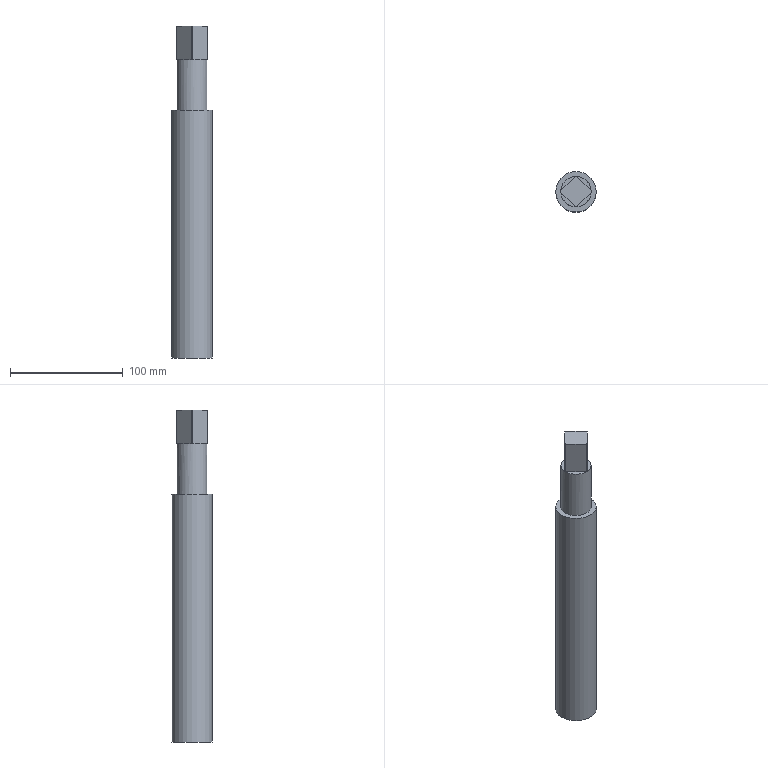Component | NX | SCREW_ROD | 1 solid | 16 faces | box 36 x 36 x 295 mm | volume 260111 mm3 | plane 12 | cylinder 3 | cone 1 | commonest cylinder face diameters 36 x1 27 x1 9.732 x1
STEP:
#1=CARTESIAN_POINT('',(0.,0.,0.));
#2=DIRECTION('',(0.,0.,1.));
#3=DIRECTION('',(1.,0.,0.));
#4=AXIS2_PLACEMENT_3D('',#1,#2,#3);
#5=CARTESIAN_POINT('',(18.,-0.,142.5));
#6=VERTEX_POINT('',#5);
#7=CARTESIAN_POINT('',(-0.,-0.,142.5));
#8=DIRECTION('',(0.,0.,1.));
#9=DIRECTION('',(1.,0.,0.));
#10=AXIS2_PLACEMENT_3D('',#7,#8,#9);
#11=CIRCLE('',#10,18.);
#12=CARTESIAN_POINT('',(-0.,-0.,142.5));
#13=DIRECTION('',(0.,0.,-1.));
#14=DIRECTION('',(-1.,0.,0.));
#15=AXIS2_PLACEMENT_3D('',#12,#13,#14);
#16=CYLINDRICAL_SURFACE('',#15,18.);
#17=CARTESIAN_POINT('',(9.425,0.));
#18=DIRECTION('',(-1.,0.));
#19=VECTOR('',#18,1.);
#20=LINE('',#17,#19);
#21=(GEOMETRIC_REPRESENTATION_CONTEXT(2)PARAMETRIC_REPRESENTATION_CONTEXT()REPRESENTATION_CONTEXT('',''));
#22=DEFINITIONAL_REPRESENTATION('',(#20),#21);
#23=PCURVE('',#16,#22);
#24=CARTESIAN_POINT('',(-0.,-0.,142.5));
#25=DIRECTION('',(0.,0.,1.));
#26=DIRECTION('',(1.,0.,0.));
#27=AXIS2_PLACEMENT_3D('',#24,#25,#26);
#28=PLANE('',#27);
#29=CARTESIAN_POINT('',(0.,0.));
#30=DIRECTION('',(1.,0.));
#31=AXIS2_PLACEMENT_2D('',#29,#30);
#32=CIRCLE('',#31,18.);
#33=(GEOMETRIC_REPRESENTATION_CONTEXT(2)PARAMETRIC_REPRESENTATION_CONTEXT()REPRESENTATION_CONTEXT('',''));
#34=DEFINITIONAL_REPRESENTATION('',(#32),#33);
#35=PCURVE('',#28,#34);
#36=SURFACE_CURVE('',#11,(#23,#35),.PCURVE_S1.);
#37=EDGE_CURVE('',#6,#6,#36,.T.);
#38=ORIENTED_EDGE('',*,*,#37,.F.);
#39=CARTESIAN_POINT('',(18.,-0.,-77.5));
#40=VERTEX_POINT('',#39);
#41=CARTESIAN_POINT('',(18.,-0.,142.5));
#42=CARTESIAN_POINT('',(18.,-0.,-77.5));
#43=B_SPLINE_CURVE_WITH_KNOTS('',1,(#41,#42),.UNSPECIFIED.,.F.,.F.,(2,2),(0.,220.),.PIECEWISE_BEZIER_KNOTS.);
#44=CARTESIAN_POINT('',(9.425,0.));
#45=DIRECTION('',(0.,1.));
#46=VECTOR('',#45,1.);
#47=LINE('',#44,#46);
#48=(GEOMETRIC_REPRESENTATION_CONTEXT(2)PARAMETRIC_REPRESENTATION_CONTEXT()REPRESENTATION_CONTEXT('',''));
#49=DEFINITIONAL_REPRESENTATION('',(#47),#48);
#50=PCURVE('',#16,#49);
#51=CARTESIAN_POINT('',(3.142,0.));
#52=DIRECTION('',(0.,1.));
#53=VECTOR('',#52,1.);
#54=LINE('',#51,#53);
#55=(GEOMETRIC_REPRESENTATION_CONTEXT(2)PARAMETRIC_REPRESENTATION_CONTEXT()REPRESENTATION_CONTEXT('',''));
#56=DEFINITIONAL_REPRESENTATION('',(#54),#55);
#57=PCURVE('',#16,#56);
#58=SEAM_CURVE('',#43,(#50,#57),.PCURVE_S1.);
#59=EDGE_CURVE('',#6,#40,#58,.T.);
#60=ORIENTED_EDGE('',*,*,#59,.T.);
#61=CARTESIAN_POINT('',(-0.,-0.,-77.5));
#62=DIRECTION('',(0.,0.,1.));
#63=DIRECTION('',(1.,0.,0.));
#64=AXIS2_PLACEMENT_3D('',#61,#62,#63);
#65=CIRCLE('',#64,18.);
#66=CARTESIAN_POINT('',(9.425,220.));
#67=DIRECTION('',(-1.,0.));
#68=VECTOR('',#67,1.);
#69=LINE('',#66,#68);
#70=(GEOMETRIC_REPRESENTATION_CONTEXT(2)PARAMETRIC_REPRESENTATION_CONTEXT()REPRESENTATION_CONTEXT('',''));
#71=DEFINITIONAL_REPRESENTATION('',(#69),#70);
#72=PCURVE('',#16,#71);
#73=CARTESIAN_POINT('',(-0.,-0.,-77.5));
#74=DIRECTION('',(0.,0.,1.));
#75=DIRECTION('',(1.,0.,0.));
#76=AXIS2_PLACEMENT_3D('',#73,#74,#75);
#77=PLANE('',#76);
#78=CARTESIAN_POINT('',(0.,0.));
#79=DIRECTION('',(1.,0.));
#80=AXIS2_PLACEMENT_2D('',#78,#79);
#81=CIRCLE('',#80,18.);
#82=(GEOMETRIC_REPRESENTATION_CONTEXT(2)PARAMETRIC_REPRESENTATION_CONTEXT()REPRESENTATION_CONTEXT('',''));
#83=DEFINITIONAL_REPRESENTATION('',(#81),#82);
#84=PCURVE('',#77,#83);
#85=SURFACE_CURVE('',#65,(#72,#84),.PCURVE_S1.);
#86=EDGE_CURVE('',#40,#40,#85,.T.);
#87=ORIENTED_EDGE('',*,*,#86,.T.);
#88=ORIENTED_EDGE('',*,*,#59,.F.);
#89=EDGE_LOOP('',(#38,#60,#87,#88));
#90=FACE_BOUND('',#89,.T.);
#91=ADVANCED_FACE('',(#90),#16,.T.);
#92=CARTESIAN_POINT('',(13.5,-0.,142.5));
#93=VERTEX_POINT('',#92);
#94=CARTESIAN_POINT('',(-13.484,-0.6582,142.5));
#95=VERTEX_POINT('',#94);
#96=CARTESIAN_POINT('',(-0.,-0.,142.5));
#97=DIRECTION('',(0.,0.,1.));
#98=DIRECTION('',(1.,0.,0.));
#99=AXIS2_PLACEMENT_3D('',#96,#97,#98);
#100=CIRCLE('',#99,13.5);
#101=CARTESIAN_POINT('',(0.,0.));
#102=DIRECTION('',(1.,0.));
#103=AXIS2_PLACEMENT_2D('',#101,#102);
#104=CIRCLE('',#103,13.5);
#105=(GEOMETRIC_REPRESENTATION_CONTEXT(2)PARAMETRIC_REPRESENTATION_CONTEXT()REPRESENTATION_CONTEXT('',''));
#106=DEFINITIONAL_REPRESENTATION('',(#104),#105);
#107=PCURVE('',#28,#106);
#108=CARTESIAN_POINT('',(-0.,-0.,217.5));
#109=DIRECTION('',(0.,0.,-1.));
#110=DIRECTION('',(-1.,0.,0.));
#111=AXIS2_PLACEMENT_3D('',#108,#109,#110);
#112=CYLINDRICAL_SURFACE('',#111,13.5);
#113=CARTESIAN_POINT('',(9.425,75.));
#114=DIRECTION('',(-1.,0.));
#115=VECTOR('',#114,1.);
#116=LINE('',#113,#115);
#117=(GEOMETRIC_REPRESENTATION_CONTEXT(2)PARAMETRIC_REPRESENTATION_CONTEXT()REPRESENTATION_CONTEXT('',''));
#118=DEFINITIONAL_REPRESENTATION('',(#116),#117);
#119=PCURVE('',#112,#118);
#120=SURFACE_CURVE('',#100,(#107,#119),.PCURVE_S1.);
#121=EDGE_CURVE('',#93,#95,#120,.T.);
#122=ORIENTED_EDGE('',*,*,#121,.F.);
#123=CARTESIAN_POINT('',(-0.,-0.,142.5));
#124=DIRECTION('',(0.,0.,1.));
#125=DIRECTION('',(1.,0.,0.));
#126=AXIS2_PLACEMENT_3D('',#123,#124,#125);
#127=CIRCLE('',#126,13.5);
#128=CARTESIAN_POINT('',(0.,0.));
#129=DIRECTION('',(1.,0.));
#130=AXIS2_PLACEMENT_2D('',#128,#129);
#131=CIRCLE('',#130,13.5);
#132=(GEOMETRIC_REPRESENTATION_CONTEXT(2)PARAMETRIC_REPRESENTATION_CONTEXT()REPRESENTATION_CONTEXT('',''));
#133=DEFINITIONAL_REPRESENTATION('',(#131),#132);
#134=PCURVE('',#28,#133);
#135=CARTESIAN_POINT('',(15.708,75.));
#136=DIRECTION('',(-1.,0.));
#137=VECTOR('',#136,1.);
#138=LINE('',#135,#137);
#139=(GEOMETRIC_REPRESENTATION_CONTEXT(2)PARAMETRIC_REPRESENTATION_CONTEXT()REPRESENTATION_CONTEXT('',''));
#140=DEFINITIONAL_REPRESENTATION('',(#138),#139);
#141=PCURVE('',#112,#140);
#142=SURFACE_CURVE('',#127,(#134,#141),.PCURVE_S1.);
#143=EDGE_CURVE('',#95,#93,#142,.T.);
#144=ORIENTED_EDGE('',*,*,#143,.F.);
#145=EDGE_LOOP('',(#122,#144));
#146=FACE_BOUND('',#145,.T.);
#147=ORIENTED_EDGE('',*,*,#37,.T.);
#148=EDGE_LOOP('',(#147));
#149=FACE_BOUND('',#148,.T.);
#150=ADVANCED_FACE('',(#146,#149),#28,.T.);
#151=CARTESIAN_POINT('',(4.866,-0.,-77.5));
#152=VERTEX_POINT('',#151);
#153=CARTESIAN_POINT('',(-0.,-0.,-77.5));
#154=DIRECTION('',(0.,0.,1.));
#155=DIRECTION('',(1.,0.,0.));
#156=AXIS2_PLACEMENT_3D('',#153,#154,#155);
#157=CIRCLE('',#156,4.866);
#158=CARTESIAN_POINT('',(0.,0.));
#159=DIRECTION('',(1.,0.));
#160=AXIS2_PLACEMENT_2D('',#158,#159);
#161=CIRCLE('',#160,4.866);
#162=(GEOMETRIC_REPRESENTATION_CONTEXT(2)PARAMETRIC_REPRESENTATION_CONTEXT()REPRESENTATION_CONTEXT('',''));
#163=DEFINITIONAL_REPRESENTATION('',(#161),#162);
#164=PCURVE('',#77,#163);
#165=CARTESIAN_POINT('',(-0.,-0.,-78.5));
#166=DIRECTION('',(0.,0.,1.));
#167=DIRECTION('',(1.,0.,0.));
#168=AXIS2_PLACEMENT_3D('',#165,#166,#167);
#169=CYLINDRICAL_SURFACE('',#168,4.866);
#170=CARTESIAN_POINT('',(0.,1.));
#171=DIRECTION('',(1.,0.));
#172=VECTOR('',#171,1.);
#173=LINE('',#170,#172);
#174=(GEOMETRIC_REPRESENTATION_CONTEXT(2)PARAMETRIC_REPRESENTATION_CONTEXT()REPRESENTATION_CONTEXT('',''));
#175=DEFINITIONAL_REPRESENTATION('',(#173),#174);
#176=PCURVE('',#169,#175);
#177=SURFACE_CURVE('',#157,(#164,#176),.PCURVE_S1.);
#178=EDGE_CURVE('',#152,#152,#177,.T.);
#179=ORIENTED_EDGE('',*,*,#178,.T.);
#180=EDGE_LOOP('',(#179));
#181=FACE_BOUND('',#180,.T.);
#182=ORIENTED_EDGE('',*,*,#86,.F.);
#183=EDGE_LOOP('',(#182));
#184=FACE_BOUND('',#183,.T.);
#185=ADVANCED_FACE('',(#181,#184),#77,.F.);
#186=CARTESIAN_POINT('',(-0.6582,-13.484,217.5));
#187=VERTEX_POINT('',#186);
#188=CARTESIAN_POINT('',(0.6582,-13.484,217.5));
#189=VERTEX_POINT('',#188);
#190=CARTESIAN_POINT('',(-0.,-0.,217.5));
#191=DIRECTION('',(0.,0.,1.));
#192=DIRECTION('',(1.,0.,0.));
#193=AXIS2_PLACEMENT_3D('',#190,#191,#192);
#194=CIRCLE('',#193,13.5);
#195=CARTESIAN_POINT('',(15.708,0.));
#196=DIRECTION('',(-1.,0.));
#197=VECTOR('',#196,1.);
#198=LINE('',#195,#197);
#199=(GEOMETRIC_REPRESENTATION_CONTEXT(2)PARAMETRIC_REPRESENTATION_CONTEXT()REPRESENTATION_CONTEXT('',''));
#200=DEFINITIONAL_REPRESENTATION('',(#198),#199);
#201=PCURVE('',#112,#200);
#202=CARTESIAN_POINT('',(-0.,-0.,217.5));
#203=DIRECTION('',(0.,0.,1.));
#204=DIRECTION('',(1.,0.,0.));
#205=AXIS2_PLACEMENT_3D('',#202,#203,#204);
#206=PLANE('',#205);
#207=CARTESIAN_POINT('',(0.,0.));
#208=DIRECTION('',(1.,0.));
#209=AXIS2_PLACEMENT_2D('',#207,#208);
#210=CIRCLE('',#209,13.5);
#211=(GEOMETRIC_REPRESENTATION_CONTEXT(2)PARAMETRIC_REPRESENTATION_CONTEXT()REPRESENTATION_CONTEXT('',''));
#212=DEFINITIONAL_REPRESENTATION('',(#210),#211);
#213=PCURVE('',#206,#212);
#214=SURFACE_CURVE('',#194,(#201,#213),.PCURVE_S1.);
#215=EDGE_CURVE('',#187,#189,#214,.T.);
#216=ORIENTED_EDGE('',*,*,#215,.F.);
#217=CARTESIAN_POINT('',(-0.6582,-13.484,187.5));
#218=VERTEX_POINT('',#217);
#219=CARTESIAN_POINT('',(-0.6582,-13.484,187.5));
#220=DIRECTION('',(0.,0.,-1.));
#221=VECTOR('',#220,1.);
#222=LINE('',#219,#221);
#223=CARTESIAN_POINT('',(11.044,30.));
#224=DIRECTION('',(0.,1.));
#225=VECTOR('',#224,1.);
#226=LINE('',#223,#225);
#227=(GEOMETRIC_REPRESENTATION_CONTEXT(2)PARAMETRIC_REPRESENTATION_CONTEXT()REPRESENTATION_CONTEXT('',''));
#228=DEFINITIONAL_REPRESENTATION('',(#226),#227);
#229=PCURVE('',#112,#228);
#230=CARTESIAN_POINT('',(-0.6582,-13.484,187.5));
#231=DIRECTION('',(0.7071,0.7071,0.));
#232=DIRECTION('',(-0.7071,0.7071,0.));
#233=AXIS2_PLACEMENT_3D('',#230,#231,#232);
#234=PLANE('',#233);
#235=CARTESIAN_POINT('',(-0.,0.));
#236=DIRECTION('',(0.,-1.));
#237=VECTOR('',#236,1.);
#238=LINE('',#235,#237);
#239=(GEOMETRIC_REPRESENTATION_CONTEXT(2)PARAMETRIC_REPRESENTATION_CONTEXT()REPRESENTATION_CONTEXT('',''));
#240=DEFINITIONAL_REPRESENTATION('',(#238),#239);
#241=PCURVE('',#234,#240);
#242=SURFACE_CURVE('',#222,(#229,#241),.PCURVE_S1.);
#243=EDGE_CURVE('',#187,#218,#242,.T.);
#244=ORIENTED_EDGE('',*,*,#243,.T.);
#245=CARTESIAN_POINT('',(-13.484,-0.6582,187.5));
#246=VERTEX_POINT('',#245);
#247=CARTESIAN_POINT('',(-0.,-0.,187.5));
#248=DIRECTION('',(0.,0.,1.));
#249=DIRECTION('',(1.,0.,0.));
#250=AXIS2_PLACEMENT_3D('',#247,#248,#249);
#251=CIRCLE('',#250,13.5);
#252=CARTESIAN_POINT('',(15.708,30.));
#253=DIRECTION('',(-1.,0.));
#254=VECTOR('',#253,1.);
#255=LINE('',#252,#254);
#256=(GEOMETRIC_REPRESENTATION_CONTEXT(2)PARAMETRIC_REPRESENTATION_CONTEXT()REPRESENTATION_CONTEXT('',''));
#257=DEFINITIONAL_REPRESENTATION('',(#255),#256);
#258=PCURVE('',#112,#257);
#259=CARTESIAN_POINT('',(-0.,-0.,187.5));
#260=DIRECTION('',(0.,0.,1.));
#261=DIRECTION('',(1.,0.,0.));
#262=AXIS2_PLACEMENT_3D('',#259,#260,#261);
#263=PLANE('',#262);
#264=CARTESIAN_POINT('',(0.,0.));
#265=DIRECTION('',(1.,0.));
#266=AXIS2_PLACEMENT_2D('',#264,#265);
#267=CIRCLE('',#266,13.5);
#268=(GEOMETRIC_REPRESENTATION_CONTEXT(2)PARAMETRIC_REPRESENTATION_CONTEXT()REPRESENTATION_CONTEXT('',''));
#269=DEFINITIONAL_REPRESENTATION('',(#267),#268);
#270=PCURVE('',#263,#269);
#271=SURFACE_CURVE('',#251,(#258,#270),.PCURVE_S1.);
#272=EDGE_CURVE('',#246,#218,#271,.T.);
#273=ORIENTED_EDGE('',*,*,#272,.F.);
#274=CARTESIAN_POINT('',(-13.484,-0.6582,187.5));
#275=CARTESIAN_POINT('',(-13.484,-0.6582,142.5));
#276=B_SPLINE_CURVE_WITH_KNOTS('',1,(#274,#275),.UNSPECIFIED.,.F.,.F.,(2,2),(30.,75.),.PIECEWISE_BEZIER_KNOTS.);
#277=CARTESIAN_POINT('',(12.518,0.));
#278=DIRECTION('',(0.,1.));
#279=VECTOR('',#278,1.);
#280=LINE('',#277,#279);
#281=(GEOMETRIC_REPRESENTATION_CONTEXT(2)PARAMETRIC_REPRESENTATION_CONTEXT()REPRESENTATION_CONTEXT('',''));
#282=DEFINITIONAL_REPRESENTATION('',(#280),#281);
#283=PCURVE('',#112,#282);
#284=CARTESIAN_POINT('',(6.234,0.));
#285=DIRECTION('',(0.,1.));
#286=VECTOR('',#285,1.);
#287=LINE('',#284,#286);
#288=(GEOMETRIC_REPRESENTATION_CONTEXT(2)PARAMETRIC_REPRESENTATION_CONTEXT()REPRESENTATION_CONTEXT('',''));
#289=DEFINITIONAL_REPRESENTATION('',(#287),#288);
#290=PCURVE('',#112,#289);
#291=SEAM_CURVE('',#276,(#283,#290),.PCURVE_S1.);
#292=EDGE_CURVE('',#246,#95,#291,.T.);
#293=ORIENTED_EDGE('',*,*,#292,.T.);
#294=ORIENTED_EDGE('',*,*,#143,.T.);
#295=ORIENTED_EDGE('',*,*,#121,.T.);
#296=ORIENTED_EDGE('',*,*,#292,.F.);
#297=CARTESIAN_POINT('',(-13.484,-0.6582,217.5));
#298=VERTEX_POINT('',#297);
#299=CARTESIAN_POINT('',(-13.484,-0.6582,187.5));
#300=DIRECTION('',(0.,0.,1.));
#301=VECTOR('',#300,1.);
#302=LINE('',#299,#301);
#303=CARTESIAN_POINT('',(6.234,30.));
#304=DIRECTION('',(0.,-1.));
#305=VECTOR('',#304,1.);
#306=LINE('',#303,#305);
#307=(GEOMETRIC_REPRESENTATION_CONTEXT(2)PARAMETRIC_REPRESENTATION_CONTEXT()REPRESENTATION_CONTEXT('',''));
#308=DEFINITIONAL_REPRESENTATION('',(#306),#307);
#309=PCURVE('',#112,#308);
#310=CARTESIAN_POINT('',(18.138,0.));
#311=DIRECTION('',(0.,1.));
#312=VECTOR('',#311,1.);
#313=LINE('',#310,#312);
#314=(GEOMETRIC_REPRESENTATION_CONTEXT(2)PARAMETRIC_REPRESENTATION_CONTEXT()REPRESENTATION_CONTEXT('',''));
#315=DEFINITIONAL_REPRESENTATION('',(#313),#314);
#316=PCURVE('',#234,#315);
#317=SURFACE_CURVE('',#302,(#309,#316),.PCURVE_S1.);
#318=EDGE_CURVE('',#246,#298,#317,.T.);
#319=ORIENTED_EDGE('',*,*,#318,.T.);
#320=CARTESIAN_POINT('',(-13.484,0.6582,217.5));
#321=VERTEX_POINT('',#320);
#322=CARTESIAN_POINT('',(-0.,-0.,217.5));
#323=DIRECTION('',(0.,0.,1.));
#324=DIRECTION('',(1.,0.,0.));
#325=AXIS2_PLACEMENT_3D('',#322,#323,#324);
#326=CIRCLE('',#325,13.5);
#327=CARTESIAN_POINT('',(9.425,0.));
#328=DIRECTION('',(-1.,0.));
#329=VECTOR('',#328,1.);
#330=LINE('',#327,#329);
#331=(GEOMETRIC_REPRESENTATION_CONTEXT(2)PARAMETRIC_REPRESENTATION_CONTEXT()REPRESENTATION_CONTEXT('',''));
#332=DEFINITIONAL_REPRESENTATION('',(#330),#331);
#333=PCURVE('',#112,#332);
#334=CARTESIAN_POINT('',(0.,0.));
#335=DIRECTION('',(1.,0.));
#336=AXIS2_PLACEMENT_2D('',#334,#335);
#337=CIRCLE('',#336,13.5);
#338=(GEOMETRIC_REPRESENTATION_CONTEXT(2)PARAMETRIC_REPRESENTATION_CONTEXT()REPRESENTATION_CONTEXT('',''));
#339=DEFINITIONAL_REPRESENTATION('',(#337),#338);
#340=PCURVE('',#206,#339);
#341=SURFACE_CURVE('',#326,(#333,#340),.PCURVE_S1.);
#342=EDGE_CURVE('',#321,#298,#341,.T.);
#343=ORIENTED_EDGE('',*,*,#342,.F.);
#344=CARTESIAN_POINT('',(-13.484,0.6582,187.5));
#345=VERTEX_POINT('',#344);
#346=CARTESIAN_POINT('',(-13.484,0.6582,187.5));
#347=DIRECTION('',(0.,0.,-1.));
#348=VECTOR('',#347,1.);
#349=LINE('',#346,#348);
#350=CARTESIAN_POINT('',(6.332,30.));
#351=DIRECTION('',(0.,1.));
#352=VECTOR('',#351,1.);
#353=LINE('',#350,#352);
#354=(GEOMETRIC_REPRESENTATION_CONTEXT(2)PARAMETRIC_REPRESENTATION_CONTEXT()REPRESENTATION_CONTEXT('',''));
#355=DEFINITIONAL_REPRESENTATION('',(#353),#354);
#356=PCURVE('',#112,#355);
#357=CARTESIAN_POINT('',(-13.484,0.6582,187.5));
#358=DIRECTION('',(0.7071,-0.7071,0.));
#359=DIRECTION('',(0.7071,0.7071,0.));
#360=AXIS2_PLACEMENT_3D('',#357,#358,#359);
#361=PLANE('',#360);
#362=CARTESIAN_POINT('',(0.,0.));
#363=DIRECTION('',(0.,-1.));
#364=VECTOR('',#363,1.);
#365=LINE('',#362,#364);
#366=(GEOMETRIC_REPRESENTATION_CONTEXT(2)PARAMETRIC_REPRESENTATION_CONTEXT()REPRESENTATION_CONTEXT('',''));
#367=DEFINITIONAL_REPRESENTATION('',(#365),#366);
#368=PCURVE('',#361,#367);
#369=SURFACE_CURVE('',#349,(#356,#368),.PCURVE_S1.);
#370=EDGE_CURVE('',#321,#345,#369,.T.);
#371=ORIENTED_EDGE('',*,*,#370,.T.);
#372=CARTESIAN_POINT('',(-0.6582,13.484,187.5));
#373=VERTEX_POINT('',#372);
#374=CARTESIAN_POINT('',(-0.,-0.,187.5));
#375=DIRECTION('',(0.,0.,1.));
#376=DIRECTION('',(1.,0.,0.));
#377=AXIS2_PLACEMENT_3D('',#374,#375,#376);
#378=CIRCLE('',#377,13.5);
#379=CARTESIAN_POINT('',(9.425,30.));
#380=DIRECTION('',(-1.,0.));
#381=VECTOR('',#380,1.);
#382=LINE('',#379,#381);
#383=(GEOMETRIC_REPRESENTATION_CONTEXT(2)PARAMETRIC_REPRESENTATION_CONTEXT()REPRESENTATION_CONTEXT('',''));
#384=DEFINITIONAL_REPRESENTATION('',(#382),#383);
#385=PCURVE('',#112,#384);
#386=CARTESIAN_POINT('',(-0.,-0.,187.5));
#387=DIRECTION('',(0.,0.,1.));
#388=DIRECTION('',(1.,0.,0.));
#389=AXIS2_PLACEMENT_3D('',#386,#387,#388);
#390=PLANE('',#389);
#391=CARTESIAN_POINT('',(0.,0.));
#392=DIRECTION('',(1.,0.));
#393=AXIS2_PLACEMENT_2D('',#391,#392);
#394=CIRCLE('',#393,13.5);
#395=(GEOMETRIC_REPRESENTATION_CONTEXT(2)PARAMETRIC_REPRESENTATION_CONTEXT()REPRESENTATION_CONTEXT('',''));
#396=DEFINITIONAL_REPRESENTATION('',(#394),#395);
#397=PCURVE('',#390,#396);
#398=SURFACE_CURVE('',#378,(#385,#397),.PCURVE_S1.);
#399=EDGE_CURVE('',#373,#345,#398,.T.);
#400=ORIENTED_EDGE('',*,*,#399,.F.);
#401=CARTESIAN_POINT('',(-0.6582,13.484,217.5));
#402=VERTEX_POINT('',#401);
#403=CARTESIAN_POINT('',(-0.6582,13.484,187.5));
#404=DIRECTION('',(0.,0.,1.));
#405=VECTOR('',#404,1.);
#406=LINE('',#403,#405);
#407=CARTESIAN_POINT('',(7.805,30.));
#408=DIRECTION('',(0.,-1.));
#409=VECTOR('',#408,1.);
#410=LINE('',#407,#409);
#411=(GEOMETRIC_REPRESENTATION_CONTEXT(2)PARAMETRIC_REPRESENTATION_CONTEXT()REPRESENTATION_CONTEXT('',''));
#412=DEFINITIONAL_REPRESENTATION('',(#410),#411);
#413=PCURVE('',#112,#412);
#414=CARTESIAN_POINT('',(18.138,0.));
#415=DIRECTION('',(0.,1.));
#416=VECTOR('',#415,1.);
#417=LINE('',#414,#416);
#418=(GEOMETRIC_REPRESENTATION_CONTEXT(2)PARAMETRIC_REPRESENTATION_CONTEXT()REPRESENTATION_CONTEXT('',''));
#419=DEFINITIONAL_REPRESENTATION('',(#417),#418);
#420=PCURVE('',#361,#419);
#421=SURFACE_CURVE('',#406,(#413,#420),.PCURVE_S1.);
#422=EDGE_CURVE('',#373,#402,#421,.T.);
#423=ORIENTED_EDGE('',*,*,#422,.T.);
#424=CARTESIAN_POINT('',(0.6582,13.484,217.5));
#425=VERTEX_POINT('',#424);
#426=CARTESIAN_POINT('',(-0.,-0.,217.5));
#427=DIRECTION('',(0.,0.,1.));
#428=DIRECTION('',(1.,0.,0.));
#429=AXIS2_PLACEMENT_3D('',#426,#427,#428);
#430=CIRCLE('',#429,13.5);
#431=CARTESIAN_POINT('',(9.425,0.));
#432=DIRECTION('',(-1.,0.));
#433=VECTOR('',#432,1.);
#434=LINE('',#431,#433);
#435=(GEOMETRIC_REPRESENTATION_CONTEXT(2)PARAMETRIC_REPRESENTATION_CONTEXT()REPRESENTATION_CONTEXT('',''));
#436=DEFINITIONAL_REPRESENTATION('',(#434),#435);
#437=PCURVE('',#112,#436);
#438=CARTESIAN_POINT('',(0.,0.));
#439=DIRECTION('',(1.,0.));
#440=AXIS2_PLACEMENT_2D('',#438,#439);
#441=CIRCLE('',#440,13.5);
#442=(GEOMETRIC_REPRESENTATION_CONTEXT(2)PARAMETRIC_REPRESENTATION_CONTEXT()REPRESENTATION_CONTEXT('',''));
#443=DEFINITIONAL_REPRESENTATION('',(#441),#442);
#444=PCURVE('',#206,#443);
#445=SURFACE_CURVE('',#430,(#437,#444),.PCURVE_S1.);
#446=EDGE_CURVE('',#425,#402,#445,.T.);
#447=ORIENTED_EDGE('',*,*,#446,.F.);
#448=CARTESIAN_POINT('',(0.6582,13.484,187.5));
#449=VERTEX_POINT('',#448);
#450=CARTESIAN_POINT('',(0.6582,13.484,187.5));
#451=DIRECTION('',(0.,0.,-1.));
#452=VECTOR('',#451,1.);
#453=LINE('',#450,#452);
#454=CARTESIAN_POINT('',(7.903,30.));
#455=DIRECTION('',(0.,1.));
#456=VECTOR('',#455,1.);
#457=LINE('',#454,#456);
#458=(GEOMETRIC_REPRESENTATION_CONTEXT(2)PARAMETRIC_REPRESENTATION_CONTEXT()REPRESENTATION_CONTEXT('',''));
#459=DEFINITIONAL_REPRESENTATION('',(#457),#458);
#460=PCURVE('',#112,#459);
#461=CARTESIAN_POINT('',(0.6582,13.484,187.5));
#462=DIRECTION('',(-0.7071,-0.7071,0.));
#463=DIRECTION('',(0.7071,-0.7071,0.));
#464=AXIS2_PLACEMENT_3D('',#461,#462,#463);
#465=PLANE('',#464);
#466=CARTESIAN_POINT('',(-0.,0.));
#467=DIRECTION('',(0.,-1.));
#468=VECTOR('',#467,1.);
#469=LINE('',#466,#468);
#470=(GEOMETRIC_REPRESENTATION_CONTEXT(2)PARAMETRIC_REPRESENTATION_CONTEXT()REPRESENTATION_CONTEXT('',''));
#471=DEFINITIONAL_REPRESENTATION('',(#469),#470);
#472=PCURVE('',#465,#471);
#473=SURFACE_CURVE('',#453,(#460,#472),.PCURVE_S1.);
#474=EDGE_CURVE('',#425,#449,#473,.T.);
#475=ORIENTED_EDGE('',*,*,#474,.T.);
#476=CARTESIAN_POINT('',(13.484,0.6582,187.5));
#477=VERTEX_POINT('',#476);
#478=CARTESIAN_POINT('',(-0.,-0.,187.5));
#479=DIRECTION('',(0.,0.,1.));
#480=DIRECTION('',(1.,0.,0.));
#481=AXIS2_PLACEMENT_3D('',#478,#479,#480);
#482=CIRCLE('',#481,13.5);
#483=CARTESIAN_POINT('',(9.425,30.));
#484=DIRECTION('',(-1.,0.));
#485=VECTOR('',#484,1.);
#486=LINE('',#483,#485);
#487=(GEOMETRIC_REPRESENTATION_CONTEXT(2)PARAMETRIC_REPRESENTATION_CONTEXT()REPRESENTATION_CONTEXT('',''));
#488=DEFINITIONAL_REPRESENTATION('',(#486),#487);
#489=PCURVE('',#112,#488);
#490=CARTESIAN_POINT('',(-0.,-0.,187.5));
#491=DIRECTION('',(0.,0.,1.));
#492=DIRECTION('',(1.,0.,0.));
#493=AXIS2_PLACEMENT_3D('',#490,#491,#492);
#494=PLANE('',#493);
#495=CARTESIAN_POINT('',(0.,0.));
#496=DIRECTION('',(1.,0.));
#497=AXIS2_PLACEMENT_2D('',#495,#496);
#498=CIRCLE('',#497,13.5);
#499=(GEOMETRIC_REPRESENTATION_CONTEXT(2)PARAMETRIC_REPRESENTATION_CONTEXT()REPRESENTATION_CONTEXT('',''));
#500=DEFINITIONAL_REPRESENTATION('',(#498),#499);
#501=PCURVE('',#494,#500);
#502=SURFACE_CURVE('',#482,(#489,#501),.PCURVE_S1.);
#503=EDGE_CURVE('',#477,#449,#502,.T.);
#504=ORIENTED_EDGE('',*,*,#503,.F.);
#505=CARTESIAN_POINT('',(13.484,0.6582,217.5));
#506=VERTEX_POINT('',#505);
#507=CARTESIAN_POINT('',(13.484,0.6582,187.5));
#508=DIRECTION('',(0.,0.,1.));
#509=VECTOR('',#508,1.);
#510=LINE('',#507,#509);
#511=CARTESIAN_POINT('',(9.376,30.));
#512=DIRECTION('',(0.,-1.));
#513=VECTOR('',#512,1.);
#514=LINE('',#511,#513);
#515=(GEOMETRIC_REPRESENTATION_CONTEXT(2)PARAMETRIC_REPRESENTATION_CONTEXT()REPRESENTATION_CONTEXT('',''));
#516=DEFINITIONAL_REPRESENTATION('',(#514),#515);
#517=PCURVE('',#112,#516);
#518=CARTESIAN_POINT('',(18.138,0.));
#519=DIRECTION('',(0.,1.));
#520=VECTOR('',#519,1.);
#521=LINE('',#518,#520);
#522=(GEOMETRIC_REPRESENTATION_CONTEXT(2)PARAMETRIC_REPRESENTATION_CONTEXT()REPRESENTATION_CONTEXT('',''));
#523=DEFINITIONAL_REPRESENTATION('',(#521),#522);
#524=PCURVE('',#465,#523);
#525=SURFACE_CURVE('',#510,(#517,#524),.PCURVE_S1.);
#526=EDGE_CURVE('',#477,#506,#525,.T.);
#527=ORIENTED_EDGE('',*,*,#526,.T.);
#528=CARTESIAN_POINT('',(13.484,-0.6582,217.5));
#529=VERTEX_POINT('',#528);
#530=CARTESIAN_POINT('',(-0.,-0.,217.5));
#531=DIRECTION('',(0.,0.,1.));
#532=DIRECTION('',(1.,0.,0.));
#533=AXIS2_PLACEMENT_3D('',#530,#531,#532);
#534=CIRCLE('',#533,13.5);
#535=CARTESIAN_POINT('',(15.708,0.));
#536=DIRECTION('',(-1.,0.));
#537=VECTOR('',#536,1.);
#538=LINE('',#535,#537);
#539=(GEOMETRIC_REPRESENTATION_CONTEXT(2)PARAMETRIC_REPRESENTATION_CONTEXT()REPRESENTATION_CONTEXT('',''));
#540=DEFINITIONAL_REPRESENTATION('',(#538),#539);
#541=PCURVE('',#112,#540);
#542=CARTESIAN_POINT('',(0.,0.));
#543=DIRECTION('',(1.,0.));
#544=AXIS2_PLACEMENT_2D('',#542,#543);
#545=CIRCLE('',#544,13.5);
#546=(GEOMETRIC_REPRESENTATION_CONTEXT(2)PARAMETRIC_REPRESENTATION_CONTEXT()REPRESENTATION_CONTEXT('',''));
#547=DEFINITIONAL_REPRESENTATION('',(#545),#546);
#548=PCURVE('',#206,#547);
#549=SURFACE_CURVE('',#534,(#541,#548),.PCURVE_S1.);
#550=EDGE_CURVE('',#529,#506,#549,.T.);
#551=ORIENTED_EDGE('',*,*,#550,.F.);
#552=CARTESIAN_POINT('',(13.484,-0.6582,187.5));
#553=VERTEX_POINT('',#552);
#554=CARTESIAN_POINT('',(13.484,-0.6582,187.5));
#555=DIRECTION('',(0.,0.,1.));
#556=VECTOR('',#555,1.);
#557=LINE('',#554,#556);
#558=CARTESIAN_POINT('',(9.474,30.));
#559=DIRECTION('',(0.,-1.));
#560=VECTOR('',#559,1.);
#561=LINE('',#558,#560);
#562=(GEOMETRIC_REPRESENTATION_CONTEXT(2)PARAMETRIC_REPRESENTATION_CONTEXT()REPRESENTATION_CONTEXT('',''));
#563=DEFINITIONAL_REPRESENTATION('',(#561),#562);
#564=PCURVE('',#112,#563);
#565=CARTESIAN_POINT('',(13.484,-0.6582,187.5));
#566=DIRECTION('',(-0.7071,0.7071,0.));
#567=DIRECTION('',(-0.7071,-0.7071,0.));
#568=AXIS2_PLACEMENT_3D('',#565,#566,#567);
#569=PLANE('',#568);
#570=CARTESIAN_POINT('',(0.,0.));
#571=DIRECTION('',(0.,1.));
#572=VECTOR('',#571,1.);
#573=LINE('',#570,#572);
#574=(GEOMETRIC_REPRESENTATION_CONTEXT(2)PARAMETRIC_REPRESENTATION_CONTEXT()REPRESENTATION_CONTEXT('',''));
#575=DEFINITIONAL_REPRESENTATION('',(#573),#574);
#576=PCURVE('',#569,#575);
#577=SURFACE_CURVE('',#557,(#564,#576),.PCURVE_S1.);
#578=EDGE_CURVE('',#553,#529,#577,.T.);
#579=ORIENTED_EDGE('',*,*,#578,.F.);
#580=CARTESIAN_POINT('',(0.6582,-13.484,187.5));
#581=VERTEX_POINT('',#580);
#582=CARTESIAN_POINT('',(-0.,-0.,187.5));
#583=DIRECTION('',(0.,0.,1.));
#584=DIRECTION('',(1.,0.,0.));
#585=AXIS2_PLACEMENT_3D('',#582,#583,#584);
#586=CIRCLE('',#585,13.5);
#587=CARTESIAN_POINT('',(15.708,30.));
#588=DIRECTION('',(-1.,0.));
#589=VECTOR('',#588,1.);
#590=LINE('',#587,#589);
#591=(GEOMETRIC_REPRESENTATION_CONTEXT(2)PARAMETRIC_REPRESENTATION_CONTEXT()REPRESENTATION_CONTEXT('',''));
#592=DEFINITIONAL_REPRESENTATION('',(#590),#591);
#593=PCURVE('',#112,#592);
#594=CARTESIAN_POINT('',(-0.,-0.,187.5));
#595=DIRECTION('',(0.,0.,1.));
#596=DIRECTION('',(1.,0.,0.));
#597=AXIS2_PLACEMENT_3D('',#594,#595,#596);
#598=PLANE('',#597);
#599=CARTESIAN_POINT('',(0.,0.));
#600=DIRECTION('',(1.,0.));
#601=AXIS2_PLACEMENT_2D('',#599,#600);
#602=CIRCLE('',#601,13.5);
#603=(GEOMETRIC_REPRESENTATION_CONTEXT(2)PARAMETRIC_REPRESENTATION_CONTEXT()REPRESENTATION_CONTEXT('',''));
#604=DEFINITIONAL_REPRESENTATION('',(#602),#603);
#605=PCURVE('',#598,#604);
#606=SURFACE_CURVE('',#586,(#593,#605),.PCURVE_S1.);
#607=EDGE_CURVE('',#581,#553,#606,.T.);
#608=ORIENTED_EDGE('',*,*,#607,.F.);
#609=CARTESIAN_POINT('',(0.6582,-13.484,187.5));
#610=DIRECTION('',(0.,0.,-1.));
#611=VECTOR('',#610,1.);
#612=LINE('',#609,#611);
#613=CARTESIAN_POINT('',(10.947,30.));
#614=DIRECTION('',(0.,1.));
#615=VECTOR('',#614,1.);
#616=LINE('',#613,#615);
#617=(GEOMETRIC_REPRESENTATION_CONTEXT(2)PARAMETRIC_REPRESENTATION_CONTEXT()REPRESENTATION_CONTEXT('',''));
#618=DEFINITIONAL_REPRESENTATION('',(#616),#617);
#619=PCURVE('',#112,#618);
#620=CARTESIAN_POINT('',(18.138,0.));
#621=DIRECTION('',(0.,-1.));
#622=VECTOR('',#621,1.);
#623=LINE('',#620,#622);
#624=(GEOMETRIC_REPRESENTATION_CONTEXT(2)PARAMETRIC_REPRESENTATION_CONTEXT()REPRESENTATION_CONTEXT('',''));
#625=DEFINITIONAL_REPRESENTATION('',(#623),#624);
#626=PCURVE('',#569,#625);
#627=SURFACE_CURVE('',#612,(#619,#626),.PCURVE_S1.);
#628=EDGE_CURVE('',#189,#581,#627,.T.);
#629=ORIENTED_EDGE('',*,*,#628,.F.);
#630=EDGE_LOOP('',(#216,#244,#273,#293,#294,#295,#296,#319,#343,#371,#400,#423,#447,#475,#504,#527,#551,#579,#608,#629));
#631=FACE_BOUND('',#630,.T.);
#632=ADVANCED_FACE('',(#631),#112,.T.);
#633=CARTESIAN_POINT('',(-0.6582,-13.484,217.5));
#634=DIRECTION('',(-0.7071,0.7071,0.));
#635=VECTOR('',#634,1.);
#636=LINE('',#633,#635);
#637=CARTESIAN_POINT('',(-0.6582,-13.484));
#638=DIRECTION('',(-0.7071,0.7071));
#639=VECTOR('',#638,1.);
#640=LINE('',#637,#639);
#641=(GEOMETRIC_REPRESENTATION_CONTEXT(2)PARAMETRIC_REPRESENTATION_CONTEXT()REPRESENTATION_CONTEXT('',''));
#642=DEFINITIONAL_REPRESENTATION('',(#640),#641);
#643=PCURVE('',#206,#642);
#644=CARTESIAN_POINT('',(0.,30.));
#645=DIRECTION('',(1.,0.));
#646=VECTOR('',#645,1.);
#647=LINE('',#644,#646);
#648=(GEOMETRIC_REPRESENTATION_CONTEXT(2)PARAMETRIC_REPRESENTATION_CONTEXT()REPRESENTATION_CONTEXT('',''));
#649=DEFINITIONAL_REPRESENTATION('',(#647),#648);
#650=PCURVE('',#234,#649);
#651=SURFACE_CURVE('',#636,(#643,#650),.PCURVE_S1.);
#652=EDGE_CURVE('',#187,#298,#651,.T.);
#653=ORIENTED_EDGE('',*,*,#652,.F.);
#654=ORIENTED_EDGE('',*,*,#215,.T.);
#655=CARTESIAN_POINT('',(13.484,-0.6582,217.5));
#656=DIRECTION('',(-0.7071,-0.7071,0.));
#657=VECTOR('',#656,1.);
#658=LINE('',#655,#657);
#659=CARTESIAN_POINT('',(13.484,-0.6582));
#660=DIRECTION('',(-0.7071,-0.7071));
#661=VECTOR('',#660,1.);
#662=LINE('',#659,#661);
#663=(GEOMETRIC_REPRESENTATION_CONTEXT(2)PARAMETRIC_REPRESENTATION_CONTEXT()REPRESENTATION_CONTEXT('',''));
#664=DEFINITIONAL_REPRESENTATION('',(#662),#663);
#665=PCURVE('',#206,#664);
#666=CARTESIAN_POINT('',(0.,30.));
#667=DIRECTION('',(1.,0.));
#668=VECTOR('',#667,1.);
#669=LINE('',#666,#668);
#670=(GEOMETRIC_REPRESENTATION_CONTEXT(2)PARAMETRIC_REPRESENTATION_CONTEXT()REPRESENTATION_CONTEXT('',''));
#671=DEFINITIONAL_REPRESENTATION('',(#669),#670);
#672=PCURVE('',#569,#671);
#673=SURFACE_CURVE('',#658,(#665,#672),.PCURVE_S1.);
#674=EDGE_CURVE('',#529,#189,#673,.T.);
#675=ORIENTED_EDGE('',*,*,#674,.F.);
#676=ORIENTED_EDGE('',*,*,#550,.T.);
#677=CARTESIAN_POINT('',(0.6582,13.484,217.5));
#678=DIRECTION('',(0.7071,-0.7071,0.));
#679=VECTOR('',#678,1.);
#680=LINE('',#677,#679);
#681=CARTESIAN_POINT('',(0.6582,13.484));
#682=DIRECTION('',(0.7071,-0.7071));
#683=VECTOR('',#682,1.);
#684=LINE('',#681,#683);
#685=(GEOMETRIC_REPRESENTATION_CONTEXT(2)PARAMETRIC_REPRESENTATION_CONTEXT()REPRESENTATION_CONTEXT('',''));
#686=DEFINITIONAL_REPRESENTATION('',(#684),#685);
#687=PCURVE('',#206,#686);
#688=CARTESIAN_POINT('',(0.,30.));
#689=DIRECTION('',(1.,0.));
#690=VECTOR('',#689,1.);
#691=LINE('',#688,#690);
#692=(GEOMETRIC_REPRESENTATION_CONTEXT(2)PARAMETRIC_REPRESENTATION_CONTEXT()REPRESENTATION_CONTEXT('',''));
#693=DEFINITIONAL_REPRESENTATION('',(#691),#692);
#694=PCURVE('',#465,#693);
#695=SURFACE_CURVE('',#680,(#687,#694),.PCURVE_S1.);
#696=EDGE_CURVE('',#425,#506,#695,.T.);
#697=ORIENTED_EDGE('',*,*,#696,.F.);
#698=ORIENTED_EDGE('',*,*,#446,.T.);
#699=CARTESIAN_POINT('',(-13.484,0.6582,217.5));
#700=DIRECTION('',(0.7071,0.7071,0.));
#701=VECTOR('',#700,1.);
#702=LINE('',#699,#701);
#703=CARTESIAN_POINT('',(-13.484,0.6582));
#704=DIRECTION('',(0.7071,0.7071));
#705=VECTOR('',#704,1.);
#706=LINE('',#703,#705);
#707=(GEOMETRIC_REPRESENTATION_CONTEXT(2)PARAMETRIC_REPRESENTATION_CONTEXT()REPRESENTATION_CONTEXT('',''));
#708=DEFINITIONAL_REPRESENTATION('',(#706),#707);
#709=PCURVE('',#206,#708);
#710=CARTESIAN_POINT('',(0.,30.));
#711=DIRECTION('',(1.,0.));
#712=VECTOR('',#711,1.);
#713=LINE('',#710,#712);
#714=(GEOMETRIC_REPRESENTATION_CONTEXT(2)PARAMETRIC_REPRESENTATION_CONTEXT()REPRESENTATION_CONTEXT('',''));
#715=DEFINITIONAL_REPRESENTATION('',(#713),#714);
#716=PCURVE('',#361,#715);
#717=SURFACE_CURVE('',#702,(#709,#716),.PCURVE_S1.);
#718=EDGE_CURVE('',#321,#402,#717,.T.);
#719=ORIENTED_EDGE('',*,*,#718,.F.);
#720=ORIENTED_EDGE('',*,*,#342,.T.);
#721=EDGE_LOOP('',(#653,#654,#675,#676,#697,#698,#719,#720));
#722=FACE_BOUND('',#721,.T.);
#723=ADVANCED_FACE('',(#722),#206,.T.);
#724=ORIENTED_EDGE('',*,*,#503,.T.);
#725=CARTESIAN_POINT('',(0.6582,13.484,187.5));
#726=DIRECTION('',(-0.7071,0.7071,0.));
#727=VECTOR('',#726,1.);
#728=LINE('',#725,#727);
#729=CARTESIAN_POINT('',(0.6582,13.484));
#730=DIRECTION('',(-0.7071,0.7071));
#731=VECTOR('',#730,1.);
#732=LINE('',#729,#731);
#733=(GEOMETRIC_REPRESENTATION_CONTEXT(2)PARAMETRIC_REPRESENTATION_CONTEXT()REPRESENTATION_CONTEXT('',''));
#734=DEFINITIONAL_REPRESENTATION('',(#732),#733);
#735=PCURVE('',#494,#734);
#736=CARTESIAN_POINT('',(0.,0.));
#737=DIRECTION('',(-1.,0.));
#738=VECTOR('',#737,1.);
#739=LINE('',#736,#738);
#740=(GEOMETRIC_REPRESENTATION_CONTEXT(2)PARAMETRIC_REPRESENTATION_CONTEXT()REPRESENTATION_CONTEXT('',''));
#741=DEFINITIONAL_REPRESENTATION('',(#739),#740);
#742=PCURVE('',#465,#741);
#743=SURFACE_CURVE('',#728,(#735,#742),.PCURVE_S1.);
#744=EDGE_CURVE('',#477,#449,#743,.T.);
#745=ORIENTED_EDGE('',*,*,#744,.F.);
#746=EDGE_LOOP('',(#724,#745));
#747=FACE_BOUND('',#746,.T.);
#748=ADVANCED_FACE('',(#747),#494,.T.);
#749=ORIENTED_EDGE('',*,*,#696,.T.);
#750=ORIENTED_EDGE('',*,*,#526,.F.);
#751=ORIENTED_EDGE('',*,*,#744,.T.);
#752=ORIENTED_EDGE('',*,*,#474,.F.);
#753=EDGE_LOOP('',(#749,#750,#751,#752));
#754=FACE_BOUND('',#753,.T.);
#755=ADVANCED_FACE('',(#754),#465,.F.);
#756=ORIENTED_EDGE('',*,*,#607,.T.);
#757=CARTESIAN_POINT('',(13.484,-0.6582,187.5));
#758=DIRECTION('',(0.7071,0.7071,0.));
#759=VECTOR('',#758,1.);
#760=LINE('',#757,#759);
#761=CARTESIAN_POINT('',(13.484,-0.6582));
#762=DIRECTION('',(0.7071,0.7071));
#763=VECTOR('',#762,1.);
#764=LINE('',#761,#763);
#765=(GEOMETRIC_REPRESENTATION_CONTEXT(2)PARAMETRIC_REPRESENTATION_CONTEXT()REPRESENTATION_CONTEXT('',''));
#766=DEFINITIONAL_REPRESENTATION('',(#764),#765);
#767=PCURVE('',#598,#766);
#768=CARTESIAN_POINT('',(0.,0.));
#769=DIRECTION('',(-1.,0.));
#770=VECTOR('',#769,1.);
#771=LINE('',#768,#770);
#772=(GEOMETRIC_REPRESENTATION_CONTEXT(2)PARAMETRIC_REPRESENTATION_CONTEXT()REPRESENTATION_CONTEXT('',''));
#773=DEFINITIONAL_REPRESENTATION('',(#771),#772);
#774=PCURVE('',#569,#773);
#775=SURFACE_CURVE('',#760,(#767,#774),.PCURVE_S1.);
#776=EDGE_CURVE('',#581,#553,#775,.T.);
#777=ORIENTED_EDGE('',*,*,#776,.F.);
#778=EDGE_LOOP('',(#756,#777));
#779=FACE_BOUND('',#778,.T.);
#780=ADVANCED_FACE('',(#779),#598,.T.);
#781=ORIENTED_EDGE('',*,*,#674,.T.);
#782=ORIENTED_EDGE('',*,*,#628,.T.);
#783=ORIENTED_EDGE('',*,*,#776,.T.);
#784=ORIENTED_EDGE('',*,*,#578,.T.);
#785=EDGE_LOOP('',(#781,#782,#783,#784));
#786=FACE_BOUND('',#785,.T.);
#787=ADVANCED_FACE('',(#786),#569,.F.);
#788=ORIENTED_EDGE('',*,*,#399,.T.);
#789=CARTESIAN_POINT('',(-13.484,0.6582,187.5));
#790=DIRECTION('',(-0.7071,-0.7071,0.));
#791=VECTOR('',#790,1.);
#792=LINE('',#789,#791);
#793=CARTESIAN_POINT('',(-13.484,0.6582));
#794=DIRECTION('',(-0.7071,-0.7071));
#795=VECTOR('',#794,1.);
#796=LINE('',#793,#795);
#797=(GEOMETRIC_REPRESENTATION_CONTEXT(2)PARAMETRIC_REPRESENTATION_CONTEXT()REPRESENTATION_CONTEXT('',''));
#798=DEFINITIONAL_REPRESENTATION('',(#796),#797);
#799=PCURVE('',#390,#798);
#800=CARTESIAN_POINT('',(0.,0.));
#801=DIRECTION('',(-1.,0.));
#802=VECTOR('',#801,1.);
#803=LINE('',#800,#802);
#804=(GEOMETRIC_REPRESENTATION_CONTEXT(2)PARAMETRIC_REPRESENTATION_CONTEXT()REPRESENTATION_CONTEXT('',''));
#805=DEFINITIONAL_REPRESENTATION('',(#803),#804);
#806=PCURVE('',#361,#805);
#807=SURFACE_CURVE('',#792,(#799,#806),.PCURVE_S1.);
#808=EDGE_CURVE('',#373,#345,#807,.T.);
#809=ORIENTED_EDGE('',*,*,#808,.F.);
#810=EDGE_LOOP('',(#788,#809));
#811=FACE_BOUND('',#810,.T.);
#812=ADVANCED_FACE('',(#811),#390,.T.);
#813=ORIENTED_EDGE('',*,*,#718,.T.);
#814=ORIENTED_EDGE('',*,*,#422,.F.);
#815=ORIENTED_EDGE('',*,*,#808,.T.);
#816=ORIENTED_EDGE('',*,*,#370,.F.);
#817=EDGE_LOOP('',(#813,#814,#815,#816));
#818=FACE_BOUND('',#817,.T.);
#819=ADVANCED_FACE('',(#818),#361,.F.);
#820=ORIENTED_EDGE('',*,*,#272,.T.);
#821=CARTESIAN_POINT('',(-0.6582,-13.484,187.5));
#822=DIRECTION('',(0.7071,-0.7071,0.));
#823=VECTOR('',#822,1.);
#824=LINE('',#821,#823);
#825=CARTESIAN_POINT('',(-0.6582,-13.484));
#826=DIRECTION('',(0.7071,-0.7071));
#827=VECTOR('',#826,1.);
#828=LINE('',#825,#827);
#829=(GEOMETRIC_REPRESENTATION_CONTEXT(2)PARAMETRIC_REPRESENTATION_CONTEXT()REPRESENTATION_CONTEXT('',''));
#830=DEFINITIONAL_REPRESENTATION('',(#828),#829);
#831=PCURVE('',#263,#830);
#832=CARTESIAN_POINT('',(0.,0.));
#833=DIRECTION('',(-1.,0.));
#834=VECTOR('',#833,1.);
#835=LINE('',#832,#834);
#836=(GEOMETRIC_REPRESENTATION_CONTEXT(2)PARAMETRIC_REPRESENTATION_CONTEXT()REPRESENTATION_CONTEXT('',''));
#837=DEFINITIONAL_REPRESENTATION('',(#835),#836);
#838=PCURVE('',#234,#837);
#839=SURFACE_CURVE('',#824,(#831,#838),.PCURVE_S1.);
#840=EDGE_CURVE('',#246,#218,#839,.T.);
#841=ORIENTED_EDGE('',*,*,#840,.F.);
#842=EDGE_LOOP('',(#820,#841));
#843=FACE_BOUND('',#842,.T.);
#844=ADVANCED_FACE('',(#843),#263,.T.);
#845=ORIENTED_EDGE('',*,*,#652,.T.);
#846=ORIENTED_EDGE('',*,*,#318,.F.);
#847=ORIENTED_EDGE('',*,*,#840,.T.);
#848=ORIENTED_EDGE('',*,*,#243,.F.);
#849=EDGE_LOOP('',(#845,#846,#847,#848));
#850=FACE_BOUND('',#849,.T.);
#851=ADVANCED_FACE('',(#850),#234,.F.);
#852=CARTESIAN_POINT('',(4.866,-0.,-57.5));
#853=VERTEX_POINT('',#852);
#854=CARTESIAN_POINT('',(-0.,-0.,-57.5));
#855=DIRECTION('',(0.,0.,1.));
#856=DIRECTION('',(1.,0.,0.));
#857=AXIS2_PLACEMENT_3D('',#854,#855,#856);
#858=CIRCLE('',#857,4.866);
#859=CARTESIAN_POINT('',(0.,21.));
#860=DIRECTION('',(1.,0.));
#861=VECTOR('',#860,1.);
#862=LINE('',#859,#861);
#863=(GEOMETRIC_REPRESENTATION_CONTEXT(2)PARAMETRIC_REPRESENTATION_CONTEXT()REPRESENTATION_CONTEXT('',''));
#864=DEFINITIONAL_REPRESENTATION('',(#862),#863);
#865=PCURVE('',#169,#864);
#866=CARTESIAN_POINT('',(-0.,-0.,-57.5));
#867=DIRECTION('',(0.,0.,1.));
#868=DIRECTION('',(1.,0.,0.));
#869=AXIS2_PLACEMENT_3D('',#866,#867,#868);
#870=PLANE('',#869);
#871=CARTESIAN_POINT('',(0.,0.));
#872=DIRECTION('',(1.,0.));
#873=AXIS2_PLACEMENT_2D('',#871,#872);
#874=CIRCLE('',#873,4.866);
#875=(GEOMETRIC_REPRESENTATION_CONTEXT(2)PARAMETRIC_REPRESENTATION_CONTEXT()REPRESENTATION_CONTEXT('',''));
#876=DEFINITIONAL_REPRESENTATION('',(#874),#875);
#877=PCURVE('',#870,#876);
#878=SURFACE_CURVE('',#858,(#865,#877),.PCURVE_S1.);
#879=EDGE_CURVE('',#853,#853,#878,.T.);
#880=ORIENTED_EDGE('',*,*,#879,.F.);
#881=CARTESIAN_POINT('',(4.866,-0.,-77.5));
#882=CARTESIAN_POINT('',(4.866,-0.,-57.5));
#883=B_SPLINE_CURVE_WITH_KNOTS('',1,(#881,#882),.UNSPECIFIED.,.F.,.F.,(2,2),(1.,21.),.PIECEWISE_BEZIER_KNOTS.);
#884=CARTESIAN_POINT('',(0.,0.));
#885=DIRECTION('',(0.,1.));
#886=VECTOR('',#885,1.);
#887=LINE('',#884,#886);
#888=(GEOMETRIC_REPRESENTATION_CONTEXT(2)PARAMETRIC_REPRESENTATION_CONTEXT()REPRESENTATION_CONTEXT('',''));
#889=DEFINITIONAL_REPRESENTATION('',(#887),#888);
#890=PCURVE('',#169,#889);
#891=CARTESIAN_POINT('',(6.283,0.));
#892=DIRECTION('',(0.,1.));
#893=VECTOR('',#892,1.);
#894=LINE('',#891,#893);
#895=(GEOMETRIC_REPRESENTATION_CONTEXT(2)PARAMETRIC_REPRESENTATION_CONTEXT()REPRESENTATION_CONTEXT('',''));
#896=DEFINITIONAL_REPRESENTATION('',(#894),#895);
#897=PCURVE('',#169,#896);
#898=SEAM_CURVE('',#883,(#890,#897),.PCURVE_S1.);
#899=EDGE_CURVE('',#152,#853,#898,.T.);
#900=ORIENTED_EDGE('',*,*,#899,.F.);
#901=ORIENTED_EDGE('',*,*,#178,.T.);
#902=ORIENTED_EDGE('',*,*,#899,.T.);
#903=EDGE_LOOP('',(#880,#900,#901,#902));
#904=FACE_BOUND('',#903,.F.);
#905=ADVANCED_FACE('',(#904),#169,.F.);
#906=ORIENTED_EDGE('',*,*,#879,.F.);
#907=EDGE_LOOP('',(#906));
#908=FACE_BOUND('',#907,.T.);
#909=CARTESIAN_POINT('',(4.25,-0.,-57.5));
#910=VERTEX_POINT('',#909);
#911=CARTESIAN_POINT('',(-4.25,-0.,-57.5));
#912=VERTEX_POINT('',#911);
#913=CARTESIAN_POINT('',(-0.,-0.,-57.5));
#914=DIRECTION('',(0.,0.,-1.));
#915=DIRECTION('',(1.,0.,0.));
#916=AXIS2_PLACEMENT_3D('',#913,#914,#915);
#917=CIRCLE('',#916,4.25);
#918=CARTESIAN_POINT('',(4.25,0.));
#919=CARTESIAN_POINT('',(4.25,-7.361));
#920=CARTESIAN_POINT('',(-2.125,-3.681));
#921=CARTESIAN_POINT('',(-8.5,-0.));
#922=CARTESIAN_POINT('',(-2.125,3.681));
#923=CARTESIAN_POINT('',(4.25,7.361));
#924=CARTESIAN_POINT('',(4.25,0.));
#925=(BOUNDED_CURVE()B_SPLINE_CURVE(2,(#918,#919,#920,#921,#922,#923,#924),.UNSPECIFIED.,.T.,.F.)B_SPLINE_CURVE_WITH_KNOTS((1,2,2,2,2,1),(-2.094,0.,2.094,4.189,6.283,8.378),.UNSPECIFIED.)CURVE()GEOMETRIC_REPRESENTATION_ITEM()RATIONAL_B_SPLINE_CURVE((1.,0.5,1.,0.5,1.,0.5,1.))REPRESENTATION_ITEM(''));
#926=(GEOMETRIC_REPRESENTATION_CONTEXT(2)PARAMETRIC_REPRESENTATION_CONTEXT()REPRESENTATION_CONTEXT('',''));
#927=DEFINITIONAL_REPRESENTATION('',(#925),#926);
#928=PCURVE('',#870,#927);
#929=CARTESIAN_POINT('',(-0.,-0.,-57.5));
#930=DIRECTION('',(0.,0.,-1.));
#931=DIRECTION('',(-1.,0.,0.));
#932=AXIS2_PLACEMENT_3D('',#929,#930,#931);
#933=CONICAL_SURFACE('',#932,4.25,1.03);
#934=CARTESIAN_POINT('',(3.142,0.));
#935=DIRECTION('',(1.,0.));
#936=VECTOR('',#935,1.);
#937=LINE('',#934,#936);
#938=(GEOMETRIC_REPRESENTATION_CONTEXT(2)PARAMETRIC_REPRESENTATION_CONTEXT()REPRESENTATION_CONTEXT('',''));
#939=DEFINITIONAL_REPRESENTATION('',(#937),#938);
#940=PCURVE('',#933,#939);
#941=SURFACE_CURVE('',#917,(#928,#940),.PCURVE_S1.);
#942=EDGE_CURVE('',#910,#912,#941,.T.);
#943=ORIENTED_EDGE('',*,*,#942,.F.);
#944=CARTESIAN_POINT('',(-0.,-0.,-57.5));
#945=DIRECTION('',(0.,0.,-1.));
#946=DIRECTION('',(1.,0.,0.));
#947=AXIS2_PLACEMENT_3D('',#944,#945,#946);
#948=CIRCLE('',#947,4.25);
#949=CARTESIAN_POINT('',(4.25,0.));
#950=CARTESIAN_POINT('',(4.25,-7.361));
#951=CARTESIAN_POINT('',(-2.125,-3.681));
#952=CARTESIAN_POINT('',(-8.5,-0.));
#953=CARTESIAN_POINT('',(-2.125,3.681));
#954=CARTESIAN_POINT('',(4.25,7.361));
#955=CARTESIAN_POINT('',(4.25,0.));
#956=(BOUNDED_CURVE()B_SPLINE_CURVE(2,(#949,#950,#951,#952,#953,#954,#955),.UNSPECIFIED.,.T.,.F.)B_SPLINE_CURVE_WITH_KNOTS((1,2,2,2,2,1),(-2.094,0.,2.094,4.189,6.283,8.378),.UNSPECIFIED.)CURVE()GEOMETRIC_REPRESENTATION_ITEM()RATIONAL_B_SPLINE_CURVE((1.,0.5,1.,0.5,1.,0.5,1.))REPRESENTATION_ITEM(''));
#957=(GEOMETRIC_REPRESENTATION_CONTEXT(2)PARAMETRIC_REPRESENTATION_CONTEXT()REPRESENTATION_CONTEXT('',''));
#958=DEFINITIONAL_REPRESENTATION('',(#956),#957);
#959=PCURVE('',#870,#958);
#960=CARTESIAN_POINT('',(-3.142,0.));
#961=DIRECTION('',(1.,0.));
#962=VECTOR('',#961,1.);
#963=LINE('',#960,#962);
#964=(GEOMETRIC_REPRESENTATION_CONTEXT(2)PARAMETRIC_REPRESENTATION_CONTEXT()REPRESENTATION_CONTEXT('',''));
#965=DEFINITIONAL_REPRESENTATION('',(#963),#964);
#966=PCURVE('',#933,#965);
#967=SURFACE_CURVE('',#948,(#959,#966),.PCURVE_S1.);
#968=EDGE_CURVE('',#912,#910,#967,.T.);
#969=ORIENTED_EDGE('',*,*,#968,.F.);
#970=EDGE_LOOP('',(#943,#969));
#971=FACE_BOUND('',#970,.T.);
#972=ADVANCED_FACE('',(#908,#971),#870,.F.);
#973=ORIENTED_EDGE('',*,*,#968,.F.);
#974=CARTESIAN_POINT('',(-0.,-0.,-54.946));
#975=VERTEX_POINT('',#974);
#976=CARTESIAN_POINT('',(-0.,-0.,-54.946));
#977=CARTESIAN_POINT('',(-4.25,-0.,-57.5));
#978=B_SPLINE_CURVE_WITH_KNOTS('',1,(#976,#977),.UNSPECIFIED.,.F.,.F.,(2,2),(-4.958,0.),.PIECEWISE_BEZIER_KNOTS.);
#979=CARTESIAN_POINT('',(0.,0.));
#980=DIRECTION('',(0.,1.));
#981=VECTOR('',#980,1.);
#982=LINE('',#979,#981);
#983=(GEOMETRIC_REPRESENTATION_CONTEXT(2)PARAMETRIC_REPRESENTATION_CONTEXT()REPRESENTATION_CONTEXT('',''));
#984=DEFINITIONAL_REPRESENTATION('',(#982),#983);
#985=PCURVE('',#933,#984);
#986=CARTESIAN_POINT('',(6.283,0.));
#987=DIRECTION('',(0.,1.));
#988=VECTOR('',#987,1.);
#989=LINE('',#986,#988);
#990=(GEOMETRIC_REPRESENTATION_CONTEXT(2)PARAMETRIC_REPRESENTATION_CONTEXT()REPRESENTATION_CONTEXT('',''));
#991=DEFINITIONAL_REPRESENTATION('',(#989),#990);
#992=PCURVE('',#933,#991);
#993=SEAM_CURVE('',#978,(#985,#992),.PCURVE_S1.);
#994=EDGE_CURVE('',#975,#912,#993,.T.);
#995=ORIENTED_EDGE('',*,*,#994,.F.);
#996=ORIENTED_EDGE('',*,*,#994,.T.);
#997=ORIENTED_EDGE('',*,*,#942,.F.);
#998=EDGE_LOOP('',(#973,#995,#996,#997));
#999=FACE_BOUND('',#998,.F.);
#1000=ADVANCED_FACE('',(#999),#933,.F.);
#1001=CLOSED_SHELL('',(#91,#150,#185,#632,#723,#748,#755,#780,#787,#812,#819,#844,#851,#905,#972,#1000));
#1002=MANIFOLD_SOLID_BREP('',#1001);
#1003=(LENGTH_UNIT()NAMED_UNIT(*)SI_UNIT(.MILLI.,.METRE.));
#1004=UNCERTAINTY_MEASURE_WITH_UNIT(LENGTH_MEASURE(0.000002),#1003,'','');
#1005=(NAMED_UNIT(*)PLANE_ANGLE_UNIT()SI_UNIT($,.RADIAN.));
#1006=(NAMED_UNIT(*)SI_UNIT($,.STERADIAN.)SOLID_ANGLE_UNIT());
#1007=(GEOMETRIC_REPRESENTATION_CONTEXT(3)GLOBAL_UNCERTAINTY_ASSIGNED_CONTEXT((#1004))GLOBAL_UNIT_ASSIGNED_CONTEXT((#1003,#1005,#1006))REPRESENTATION_CONTEXT('',''));
#1008=ADVANCED_BREP_SHAPE_REPRESENTATION('',(#4,#1002),#1007);